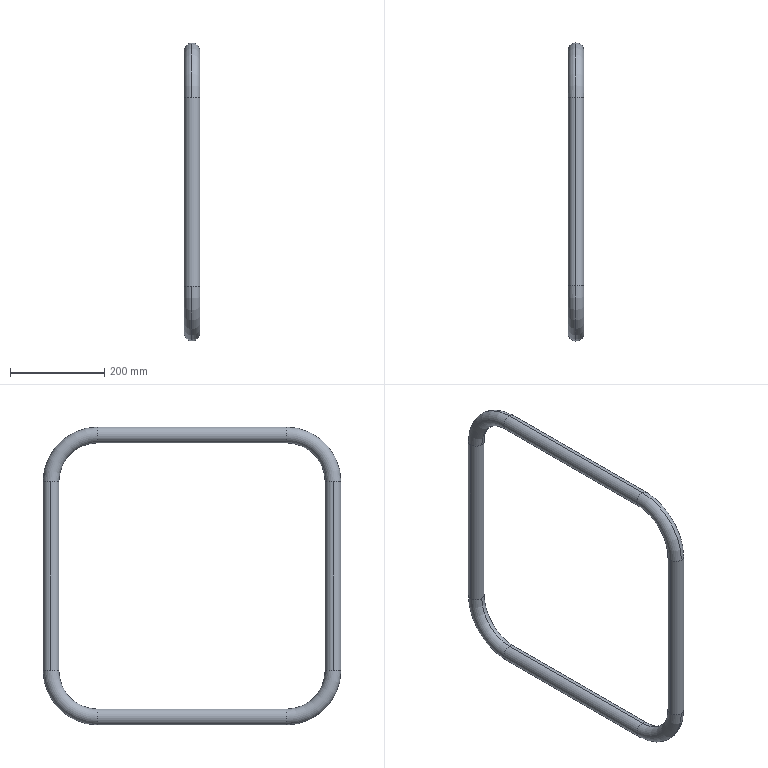Component | SolidWorks | Door-2 | 1 solid | 32 faces | box 33.5 x 633.5 x 633.5 mm | volume 640543 mm3 | torus 16 | cylinder 16 | commonest cylinder face diameters 33.5 x8 27.5 x8 | material Plain Carbon Steel
build123d program:
from build123d import *

# Parameters (mm, degrees)
SWEEP_THIN1_PROFILE_R   = 16.75
SWEEP_THIN1_PROFILE_R_2 = 13.75


with BuildPart() as part:
    # Sweep-Thin1: sweep along a path in Sketch1
    with BuildLine(Plane(origin=(0, 0, 0), x_dir=(0, 0, -1), z_dir=(1, 0, 0))) as sweep_thin1_path:
        Line((-438.875, 448.577), (-38.875, 448.577))
        ThreePointArc((-38.875, 448.577), (31.836, 419.288), (61.125, 348.577))
        Line((61.125, 348.577), (61.125, -51.423))
        ThreePointArc((61.125, -51.423), (31.836, -122.134), (-38.875, -151.423))
        Line((-38.875, -151.423), (-438.875, -151.423))
        ThreePointArc((-438.875, -151.423), (-509.586, -122.134), (-538.875, -51.423))
        Line((-538.875, -51.423), (-538.875, 348.577))
        ThreePointArc((-538.875, 348.577), (-509.586, 419.288), (-438.875, 448.577))
    # Sweep-Thin1 profile (on start of the path) → Sweep-Thin1 (sweep)
    with BuildSketch(Plane(origin=(0, 448.577, 438.875), x_dir=(-1, 0, 0), z_dir=(0, 0, -1))):
        Circle(SWEEP_THIN1_PROFILE_R)
        Circle(SWEEP_THIN1_PROFILE_R_2, mode=Mode.SUBTRACT)
    sweep(path=sweep_thin1_path.line)


solid = part.part

# Placed as in the assembly
solid = solid.moved(Location((-3322.199, 2439.746, 6247.098), (0, 0, 0)))
STEP:
#1=COLOUR_RGB('',0.7922,0.8196,0.9333);
#2=FILL_AREA_STYLE_COLOUR('',#1);
#3=FILL_AREA_STYLE('',(#2));
#4=SURFACE_STYLE_FILL_AREA(#3);
#5=SURFACE_SIDE_STYLE('',(#4));
#6=SURFACE_STYLE_USAGE(.BOTH.,#5);
#7=PRESENTATION_STYLE_ASSIGNMENT((#6));
#8=CARTESIAN_POINT('',(-130.795,89.432,263.227));
#9=VERTEX_POINT('',#8);
#10=CARTESIAN_POINT('',(-131.455,90.091,263.227));
#11=VERTEX_POINT('',#10);
#12=CARTESIAN_POINT('',(-130.795,90.091,263.227));
#13=DIRECTION('',(0.,0.,-1.));
#14=DIRECTION('',(0.,1.,0.));
#15=AXIS2_PLACEMENT_3D('',#12,#13,#14);
#16=CIRCLE('',#15,0.6594);
#17=EDGE_CURVE('',#9,#11,#16,.T.);
#18=ORIENTED_EDGE('',*,*,#17,.F.);
#19=CARTESIAN_POINT('',(-130.795,94.028,267.824));
#20=VERTEX_POINT('',#19);
#21=CARTESIAN_POINT('',(-130.795,94.028,263.227));
#22=DIRECTION('',(-1.,0.,0.));
#23=DIRECTION('',(0.,0.,1.));
#24=AXIS2_PLACEMENT_3D('',#21,#22,#23);
#25=CIRCLE('',#24,4.596);
#26=EDGE_CURVE('',#9,#20,#25,.T.);
#27=ORIENTED_EDGE('',*,*,#26,.T.);
#28=CARTESIAN_POINT('',(-130.795,94.028,266.505));
#29=VERTEX_POINT('',#28);
#30=CARTESIAN_POINT('',(-130.795,94.028,267.164));
#31=DIRECTION('',(0.,-1.,-0.));
#32=DIRECTION('',(0.,0.,-1.));
#33=AXIS2_PLACEMENT_3D('',#30,#31,#32);
#34=CIRCLE('',#33,0.6594);
#35=EDGE_CURVE('',#20,#29,#34,.T.);
#36=ORIENTED_EDGE('',*,*,#35,.T.);
#37=CARTESIAN_POINT('',(-130.795,90.751,263.227));
#38=VERTEX_POINT('',#37);
#39=CARTESIAN_POINT('',(-130.795,94.028,263.227));
#40=DIRECTION('',(-1.,0.,0.));
#41=DIRECTION('',(0.,0.,1.));
#42=AXIS2_PLACEMENT_3D('',#39,#40,#41);
#43=CIRCLE('',#42,3.278);
#44=EDGE_CURVE('',#38,#29,#43,.T.);
#45=ORIENTED_EDGE('',*,*,#44,.F.);
#46=CARTESIAN_POINT('',(-130.795,90.091,263.227));
#47=DIRECTION('',(0.,0.,-1.));
#48=DIRECTION('',(0.,1.,0.));
#49=AXIS2_PLACEMENT_3D('',#46,#47,#48);
#50=CIRCLE('',#49,0.6594);
#51=EDGE_CURVE('',#11,#38,#50,.T.);
#52=ORIENTED_EDGE('',*,*,#51,.F.);
#53=EDGE_LOOP('',(#18,#27,#36,#45,#52));
#54=FACE_OUTER_BOUND('',#53,.T.);
#55=CARTESIAN_POINT('',(-130.795,94.028,263.227));
#56=DIRECTION('',(-1.,0.,0.));
#57=DIRECTION('',(0.,0.,1.));
#58=AXIS2_PLACEMENT_3D('',#55,#56,#57);
#59=TOROIDAL_SURFACE('',#58,3.937,0.6594);
#60=ADVANCED_FACE('',(#54),#59,.T.);
#61=CARTESIAN_POINT('',(-130.795,94.028,242.883));
#62=VERTEX_POINT('',#61);
#63=CARTESIAN_POINT('',(-130.795,94.028,244.202));
#64=VERTEX_POINT('',#63);
#65=CARTESIAN_POINT('',(-130.795,94.028,243.542));
#66=DIRECTION('',(0.,1.,0.));
#67=DIRECTION('',(0.,0.,1.));
#68=AXIS2_PLACEMENT_3D('',#65,#66,#67);
#69=CIRCLE('',#68,0.6594);
#70=EDGE_CURVE('',#62,#64,#69,.T.);
#71=ORIENTED_EDGE('',*,*,#70,.F.);
#72=CARTESIAN_POINT('',(-130.795,89.432,247.479));
#73=VERTEX_POINT('',#72);
#74=CARTESIAN_POINT('',(-130.795,94.028,247.479));
#75=DIRECTION('',(-1.,0.,0.));
#76=DIRECTION('',(0.,0.,1.));
#77=AXIS2_PLACEMENT_3D('',#74,#75,#76);
#78=CIRCLE('',#77,4.596);
#79=EDGE_CURVE('',#62,#73,#78,.T.);
#80=ORIENTED_EDGE('',*,*,#79,.T.);
#81=CARTESIAN_POINT('',(-131.455,90.091,247.479));
#82=VERTEX_POINT('',#81);
#83=CARTESIAN_POINT('',(-130.795,90.091,247.479));
#84=DIRECTION('',(0.,0.,-1.));
#85=DIRECTION('',(0.,1.,0.));
#86=AXIS2_PLACEMENT_3D('',#83,#84,#85);
#87=CIRCLE('',#86,0.6594);
#88=EDGE_CURVE('',#73,#82,#87,.T.);
#89=ORIENTED_EDGE('',*,*,#88,.T.);
#90=CARTESIAN_POINT('',(-130.795,90.751,247.479));
#91=VERTEX_POINT('',#90);
#92=CARTESIAN_POINT('',(-130.795,90.091,247.479));
#93=DIRECTION('',(0.,0.,-1.));
#94=DIRECTION('',(0.,1.,0.));
#95=AXIS2_PLACEMENT_3D('',#92,#93,#94);
#96=CIRCLE('',#95,0.6594);
#97=EDGE_CURVE('',#82,#91,#96,.T.);
#98=ORIENTED_EDGE('',*,*,#97,.T.);
#99=CARTESIAN_POINT('',(-130.795,94.028,247.479));
#100=DIRECTION('',(-1.,0.,0.));
#101=DIRECTION('',(0.,0.,1.));
#102=AXIS2_PLACEMENT_3D('',#99,#100,#101);
#103=CIRCLE('',#102,3.278);
#104=EDGE_CURVE('',#64,#91,#103,.T.);
#105=ORIENTED_EDGE('',*,*,#104,.F.);
#106=EDGE_LOOP('',(#71,#80,#89,#98,#105));
#107=FACE_OUTER_BOUND('',#106,.T.);
#108=CARTESIAN_POINT('',(-130.795,94.028,247.479));
#109=DIRECTION('',(-1.,0.,0.));
#110=DIRECTION('',(0.,0.,1.));
#111=AXIS2_PLACEMENT_3D('',#108,#109,#110);
#112=TOROIDAL_SURFACE('',#111,3.937,0.6594);
#113=ADVANCED_FACE('',(#107),#112,.T.);
#114=CARTESIAN_POINT('',(-130.795,114.373,247.479));
#115=VERTEX_POINT('',#114);
#116=CARTESIAN_POINT('',(-131.455,113.713,247.479));
#117=VERTEX_POINT('',#116);
#118=CARTESIAN_POINT('',(-130.795,113.713,247.479));
#119=DIRECTION('',(0.,-0.,1.));
#120=DIRECTION('',(0.,-1.,0.));
#121=AXIS2_PLACEMENT_3D('',#118,#119,#120);
#122=CIRCLE('',#121,0.6594);
#123=EDGE_CURVE('',#115,#117,#122,.T.);
#124=ORIENTED_EDGE('',*,*,#123,.F.);
#125=CARTESIAN_POINT('',(-130.795,109.776,242.883));
#126=VERTEX_POINT('',#125);
#127=CARTESIAN_POINT('',(-130.795,109.776,247.479));
#128=DIRECTION('',(-1.,0.,0.));
#129=DIRECTION('',(0.,0.,1.));
#130=AXIS2_PLACEMENT_3D('',#127,#128,#129);
#131=CIRCLE('',#130,4.596);
#132=EDGE_CURVE('',#115,#126,#131,.T.);
#133=ORIENTED_EDGE('',*,*,#132,.T.);
#134=CARTESIAN_POINT('',(-130.795,109.776,244.202));
#135=VERTEX_POINT('',#134);
#136=CARTESIAN_POINT('',(-130.795,109.776,243.542));
#137=DIRECTION('',(0.,1.,0.));
#138=DIRECTION('',(0.,0.,1.));
#139=AXIS2_PLACEMENT_3D('',#136,#137,#138);
#140=CIRCLE('',#139,0.6594);
#141=EDGE_CURVE('',#126,#135,#140,.T.);
#142=ORIENTED_EDGE('',*,*,#141,.T.);
#143=CARTESIAN_POINT('',(-130.795,113.054,247.479));
#144=VERTEX_POINT('',#143);
#145=CARTESIAN_POINT('',(-130.795,109.776,247.479));
#146=DIRECTION('',(-1.,0.,0.));
#147=DIRECTION('',(0.,0.,1.));
#148=AXIS2_PLACEMENT_3D('',#145,#146,#147);
#149=CIRCLE('',#148,3.278);
#150=EDGE_CURVE('',#144,#135,#149,.T.);
#151=ORIENTED_EDGE('',*,*,#150,.F.);
#152=CARTESIAN_POINT('',(-130.795,113.713,247.479));
#153=DIRECTION('',(0.,-0.,1.));
#154=DIRECTION('',(0.,-1.,0.));
#155=AXIS2_PLACEMENT_3D('',#152,#153,#154);
#156=CIRCLE('',#155,0.6594);
#157=EDGE_CURVE('',#117,#144,#156,.T.);
#158=ORIENTED_EDGE('',*,*,#157,.F.);
#159=EDGE_LOOP('',(#124,#133,#142,#151,#158));
#160=FACE_OUTER_BOUND('',#159,.T.);
#161=CARTESIAN_POINT('',(-130.795,109.776,247.479));
#162=DIRECTION('',(-1.,0.,0.));
#163=DIRECTION('',(0.,0.,1.));
#164=AXIS2_PLACEMENT_3D('',#161,#162,#163);
#165=TOROIDAL_SURFACE('',#164,3.937,0.6594);
#166=ADVANCED_FACE('',(#160),#165,.T.);
#167=CARTESIAN_POINT('',(-130.795,109.776,267.824));
#168=VERTEX_POINT('',#167);
#169=CARTESIAN_POINT('',(-130.795,109.776,266.505));
#170=VERTEX_POINT('',#169);
#171=CARTESIAN_POINT('',(-130.795,109.776,267.164));
#172=DIRECTION('',(0.,-1.,-0.));
#173=DIRECTION('',(0.,0.,-1.));
#174=AXIS2_PLACEMENT_3D('',#171,#172,#173);
#175=CIRCLE('',#174,0.6594);
#176=EDGE_CURVE('',#168,#170,#175,.T.);
#177=ORIENTED_EDGE('',*,*,#176,.F.);
#178=CARTESIAN_POINT('',(-130.795,114.373,263.227));
#179=VERTEX_POINT('',#178);
#180=CARTESIAN_POINT('',(-130.795,109.776,263.227));
#181=DIRECTION('',(-1.,0.,0.));
#182=DIRECTION('',(0.,0.,1.));
#183=AXIS2_PLACEMENT_3D('',#180,#181,#182);
#184=CIRCLE('',#183,4.596);
#185=EDGE_CURVE('',#168,#179,#184,.T.);
#186=ORIENTED_EDGE('',*,*,#185,.T.);
#187=CARTESIAN_POINT('',(-131.455,113.713,263.227));
#188=VERTEX_POINT('',#187);
#189=CARTESIAN_POINT('',(-130.795,113.713,263.227));
#190=DIRECTION('',(0.,-0.,1.));
#191=DIRECTION('',(0.,-1.,0.));
#192=AXIS2_PLACEMENT_3D('',#189,#190,#191);
#193=CIRCLE('',#192,0.6594);
#194=EDGE_CURVE('',#179,#188,#193,.T.);
#195=ORIENTED_EDGE('',*,*,#194,.T.);
#196=CARTESIAN_POINT('',(-130.795,113.054,263.227));
#197=VERTEX_POINT('',#196);
#198=CARTESIAN_POINT('',(-130.795,113.713,263.227));
#199=DIRECTION('',(0.,-0.,1.));
#200=DIRECTION('',(0.,-1.,0.));
#201=AXIS2_PLACEMENT_3D('',#198,#199,#200);
#202=CIRCLE('',#201,0.6594);
#203=EDGE_CURVE('',#188,#197,#202,.T.);
#204=ORIENTED_EDGE('',*,*,#203,.T.);
#205=CARTESIAN_POINT('',(-130.795,109.776,263.227));
#206=DIRECTION('',(-1.,0.,0.));
#207=DIRECTION('',(0.,0.,1.));
#208=AXIS2_PLACEMENT_3D('',#205,#206,#207);
#209=CIRCLE('',#208,3.278);
#210=EDGE_CURVE('',#170,#197,#209,.T.);
#211=ORIENTED_EDGE('',*,*,#210,.F.);
#212=EDGE_LOOP('',(#177,#186,#195,#204,#211));
#213=FACE_OUTER_BOUND('',#212,.T.);
#214=CARTESIAN_POINT('',(-130.795,109.776,263.227));
#215=DIRECTION('',(-1.,0.,0.));
#216=DIRECTION('',(0.,0.,1.));
#217=AXIS2_PLACEMENT_3D('',#214,#215,#216);
#218=TOROIDAL_SURFACE('',#217,3.937,0.6594);
#219=ADVANCED_FACE('',(#213),#218,.T.);
#220=CARTESIAN_POINT('',(-130.795,94.028,267.164));
#221=DIRECTION('',(0.,-1.,-0.));
#222=DIRECTION('',(0.,0.,-1.));
#223=AXIS2_PLACEMENT_3D('',#220,#221,#222);
#224=CIRCLE('',#223,0.6594);
#225=EDGE_CURVE('',#29,#20,#224,.T.);
#226=ORIENTED_EDGE('',*,*,#225,.F.);
#227=CARTESIAN_POINT('',(-130.795,94.028,266.505));
#228=DIRECTION('',(0.,1.,0.));
#229=VECTOR('',#228,39.37);
#230=LINE('',#227,#229);
#231=EDGE_CURVE('',#29,#170,#230,.T.);
#232=ORIENTED_EDGE('',*,*,#231,.T.);
#233=CARTESIAN_POINT('',(-130.795,109.776,267.164));
#234=DIRECTION('',(0.,-1.,-0.));
#235=DIRECTION('',(0.,0.,-1.));
#236=AXIS2_PLACEMENT_3D('',#233,#234,#235);
#237=CIRCLE('',#236,0.6594);
#238=EDGE_CURVE('',#170,#168,#237,.T.);
#239=ORIENTED_EDGE('',*,*,#238,.T.);
#240=CARTESIAN_POINT('',(-130.795,94.028,267.824));
#241=DIRECTION('',(0.,1.,0.));
#242=VECTOR('',#241,39.37);
#243=LINE('',#240,#242);
#244=EDGE_CURVE('',#20,#168,#243,.T.);
#245=ORIENTED_EDGE('',*,*,#244,.F.);
#246=EDGE_LOOP('',(#226,#232,#239,#245));
#247=FACE_OUTER_BOUND('',#246,.T.);
#248=CARTESIAN_POINT('',(-130.795,94.028,267.164));
#249=DIRECTION('',(0.,1.,0.));
#250=DIRECTION('',(0.,0.,1.));
#251=AXIS2_PLACEMENT_3D('',#248,#249,#250);
#252=CYLINDRICAL_SURFACE('',#251,0.6594);
#253=ADVANCED_FACE('',(#247),#252,.T.);
#254=ORIENTED_EDGE('',*,*,#97,.F.);
#255=CARTESIAN_POINT('',(-131.455,90.091,247.479));
#256=DIRECTION('',(0.,0.,1.));
#257=VECTOR('',#256,39.37);
#258=LINE('',#255,#257);
#259=EDGE_CURVE('',#82,#11,#258,.T.);
#260=ORIENTED_EDGE('',*,*,#259,.T.);
#261=ORIENTED_EDGE('',*,*,#51,.T.);
#262=CARTESIAN_POINT('',(-130.136,90.091,263.227));
#263=VERTEX_POINT('',#262);
#264=CARTESIAN_POINT('',(-130.795,90.091,263.227));
#265=DIRECTION('',(0.,0.,-1.));
#266=DIRECTION('',(0.,1.,0.));
#267=AXIS2_PLACEMENT_3D('',#264,#265,#266);
#268=CIRCLE('',#267,0.6594);
#269=EDGE_CURVE('',#38,#263,#268,.T.);
#270=ORIENTED_EDGE('',*,*,#269,.T.);
#271=CARTESIAN_POINT('',(-130.136,90.091,247.479));
#272=VERTEX_POINT('',#271);
#273=CARTESIAN_POINT('',(-130.136,90.091,247.479));
#274=DIRECTION('',(0.,0.,1.));
#275=VECTOR('',#274,39.37);
#276=LINE('',#273,#275);
#277=EDGE_CURVE('',#272,#263,#276,.T.);
#278=ORIENTED_EDGE('',*,*,#277,.F.);
#279=CARTESIAN_POINT('',(-130.795,90.091,247.479));
#280=DIRECTION('',(0.,0.,-1.));
#281=DIRECTION('',(0.,1.,0.));
#282=AXIS2_PLACEMENT_3D('',#279,#280,#281);
#283=CIRCLE('',#282,0.6594);
#284=EDGE_CURVE('',#91,#272,#283,.T.);
#285=ORIENTED_EDGE('',*,*,#284,.F.);
#286=EDGE_LOOP('',(#254,#260,#261,#270,#278,#285));
#287=FACE_OUTER_BOUND('',#286,.T.);
#288=CARTESIAN_POINT('',(-130.795,90.091,247.479));
#289=DIRECTION('',(0.,0.,1.));
#290=DIRECTION('',(1.,0.,0.));
#291=AXIS2_PLACEMENT_3D('',#288,#289,#290);
#292=CYLINDRICAL_SURFACE('',#291,0.6594);
#293=ADVANCED_FACE('',(#287),#292,.T.);
#294=CARTESIAN_POINT('',(-130.795,109.776,243.542));
#295=DIRECTION('',(0.,1.,0.));
#296=DIRECTION('',(0.,0.,1.));
#297=AXIS2_PLACEMENT_3D('',#294,#295,#296);
#298=CIRCLE('',#297,0.6594);
#299=EDGE_CURVE('',#135,#126,#298,.T.);
#300=ORIENTED_EDGE('',*,*,#299,.F.);
#301=CARTESIAN_POINT('',(-130.795,109.776,244.202));
#302=DIRECTION('',(0.,-1.,-0.));
#303=VECTOR('',#302,39.37);
#304=LINE('',#301,#303);
#305=EDGE_CURVE('',#135,#64,#304,.T.);
#306=ORIENTED_EDGE('',*,*,#305,.T.);
#307=CARTESIAN_POINT('',(-130.795,94.028,243.542));
#308=DIRECTION('',(0.,1.,0.));
#309=DIRECTION('',(0.,0.,1.));
#310=AXIS2_PLACEMENT_3D('',#307,#308,#309);
#311=CIRCLE('',#310,0.6594);
#312=EDGE_CURVE('',#64,#62,#311,.T.);
#313=ORIENTED_EDGE('',*,*,#312,.T.);
#314=CARTESIAN_POINT('',(-130.795,109.776,242.883));
#315=DIRECTION('',(0.,-1.,-0.));
#316=VECTOR('',#315,39.37);
#317=LINE('',#314,#316);
#318=EDGE_CURVE('',#126,#62,#317,.T.);
#319=ORIENTED_EDGE('',*,*,#318,.F.);
#320=EDGE_LOOP('',(#300,#306,#313,#319));
#321=FACE_OUTER_BOUND('',#320,.T.);
#322=CARTESIAN_POINT('',(-130.795,109.776,243.542));
#323=DIRECTION('',(0.,-1.,-0.));
#324=DIRECTION('',(0.,0.,-1.));
#325=AXIS2_PLACEMENT_3D('',#322,#323,#324);
#326=CYLINDRICAL_SURFACE('',#325,0.6594);
#327=ADVANCED_FACE('',(#321),#326,.T.);
#328=CARTESIAN_POINT('',(-130.136,113.713,263.227));
#329=VERTEX_POINT('',#328);
#330=CARTESIAN_POINT('',(-130.795,113.713,263.227));
#331=DIRECTION('',(0.,-0.,1.));
#332=DIRECTION('',(0.,-1.,0.));
#333=AXIS2_PLACEMENT_3D('',#330,#331,#332);
#334=CIRCLE('',#333,0.6594);
#335=EDGE_CURVE('',#329,#179,#334,.T.);
#336=ORIENTED_EDGE('',*,*,#335,.F.);
#337=CARTESIAN_POINT('',(-130.136,113.713,247.479));
#338=VERTEX_POINT('',#337);
#339=CARTESIAN_POINT('',(-130.136,113.713,263.227));
#340=DIRECTION('',(0.,0.,-1.));
#341=VECTOR('',#340,39.37);
#342=LINE('',#339,#341);
#343=EDGE_CURVE('',#329,#338,#342,.T.);
#344=ORIENTED_EDGE('',*,*,#343,.T.);
#345=CARTESIAN_POINT('',(-130.795,113.713,247.479));
#346=DIRECTION('',(0.,-0.,1.));
#347=DIRECTION('',(0.,-1.,0.));
#348=AXIS2_PLACEMENT_3D('',#345,#346,#347);
#349=CIRCLE('',#348,0.6594);
#350=EDGE_CURVE('',#338,#115,#349,.T.);
#351=ORIENTED_EDGE('',*,*,#350,.T.);
#352=ORIENTED_EDGE('',*,*,#123,.T.);
#353=CARTESIAN_POINT('',(-131.455,113.713,263.227));
#354=DIRECTION('',(0.,0.,-1.));
#355=VECTOR('',#354,39.37);
#356=LINE('',#353,#355);
#357=EDGE_CURVE('',#188,#117,#356,.T.);
#358=ORIENTED_EDGE('',*,*,#357,.F.);
#359=ORIENTED_EDGE('',*,*,#194,.F.);
#360=EDGE_LOOP('',(#336,#344,#351,#352,#358,#359));
#361=FACE_OUTER_BOUND('',#360,.T.);
#362=CARTESIAN_POINT('',(-130.795,113.713,263.227));
#363=DIRECTION('',(0.,0.,-1.));
#364=DIRECTION('',(-1.,0.,0.));
#365=AXIS2_PLACEMENT_3D('',#362,#363,#364);
#366=CYLINDRICAL_SURFACE('',#365,0.6594);
#367=ADVANCED_FACE('',(#361),#366,.T.);
#368=ORIENTED_EDGE('',*,*,#185,.F.);
#369=ORIENTED_EDGE('',*,*,#238,.F.);
#370=ORIENTED_EDGE('',*,*,#210,.T.);
#371=CARTESIAN_POINT('',(-130.795,113.713,263.227));
#372=DIRECTION('',(0.,-0.,1.));
#373=DIRECTION('',(0.,-1.,0.));
#374=AXIS2_PLACEMENT_3D('',#371,#372,#373);
#375=CIRCLE('',#374,0.6594);
#376=EDGE_CURVE('',#197,#329,#375,.T.);
#377=ORIENTED_EDGE('',*,*,#376,.T.);
#378=ORIENTED_EDGE('',*,*,#335,.T.);
#379=EDGE_LOOP('',(#368,#369,#370,#377,#378));
#380=FACE_OUTER_BOUND('',#379,.T.);
#381=CARTESIAN_POINT('',(-130.795,109.776,263.227));
#382=DIRECTION('',(-1.,0.,0.));
#383=DIRECTION('',(0.,0.,1.));
#384=AXIS2_PLACEMENT_3D('',#381,#382,#383);
#385=TOROIDAL_SURFACE('',#384,3.937,0.6594);
#386=ADVANCED_FACE('',(#380),#385,.T.);
#387=ORIENTED_EDGE('',*,*,#343,.F.);
#388=ORIENTED_EDGE('',*,*,#376,.F.);
#389=ORIENTED_EDGE('',*,*,#203,.F.);
#390=ORIENTED_EDGE('',*,*,#357,.T.);
#391=ORIENTED_EDGE('',*,*,#157,.T.);
#392=CARTESIAN_POINT('',(-130.795,113.713,247.479));
#393=DIRECTION('',(0.,-0.,1.));
#394=DIRECTION('',(0.,-1.,0.));
#395=AXIS2_PLACEMENT_3D('',#392,#393,#394);
#396=CIRCLE('',#395,0.6594);
#397=EDGE_CURVE('',#144,#338,#396,.T.);
#398=ORIENTED_EDGE('',*,*,#397,.T.);
#399=EDGE_LOOP('',(#387,#388,#389,#390,#391,#398));
#400=FACE_OUTER_BOUND('',#399,.T.);
#401=CARTESIAN_POINT('',(-130.795,113.713,263.227));
#402=DIRECTION('',(0.,0.,-1.));
#403=DIRECTION('',(-1.,0.,0.));
#404=AXIS2_PLACEMENT_3D('',#401,#402,#403);
#405=CYLINDRICAL_SURFACE('',#404,0.6594);
#406=ADVANCED_FACE('',(#400),#405,.T.);
#407=ORIENTED_EDGE('',*,*,#132,.F.);
#408=ORIENTED_EDGE('',*,*,#350,.F.);
#409=ORIENTED_EDGE('',*,*,#397,.F.);
#410=ORIENTED_EDGE('',*,*,#150,.T.);
#411=ORIENTED_EDGE('',*,*,#299,.T.);
#412=EDGE_LOOP('',(#407,#408,#409,#410,#411));
#413=FACE_OUTER_BOUND('',#412,.T.);
#414=CARTESIAN_POINT('',(-130.795,109.776,247.479));
#415=DIRECTION('',(-1.,0.,0.));
#416=DIRECTION('',(0.,0.,1.));
#417=AXIS2_PLACEMENT_3D('',#414,#415,#416);
#418=TOROIDAL_SURFACE('',#417,3.937,0.6594);
#419=ADVANCED_FACE('',(#413),#418,.T.);
#420=ORIENTED_EDGE('',*,*,#305,.F.);
#421=ORIENTED_EDGE('',*,*,#141,.F.);
#422=ORIENTED_EDGE('',*,*,#318,.T.);
#423=ORIENTED_EDGE('',*,*,#70,.T.);
#424=EDGE_LOOP('',(#420,#421,#422,#423));
#425=FACE_OUTER_BOUND('',#424,.T.);
#426=CARTESIAN_POINT('',(-130.795,109.776,243.542));
#427=DIRECTION('',(0.,-1.,-0.));
#428=DIRECTION('',(0.,0.,-1.));
#429=AXIS2_PLACEMENT_3D('',#426,#427,#428);
#430=CYLINDRICAL_SURFACE('',#429,0.6594);
#431=ADVANCED_FACE('',(#425),#430,.T.);
#432=ORIENTED_EDGE('',*,*,#79,.F.);
#433=ORIENTED_EDGE('',*,*,#312,.F.);
#434=ORIENTED_EDGE('',*,*,#104,.T.);
#435=ORIENTED_EDGE('',*,*,#284,.T.);
#436=CARTESIAN_POINT('',(-130.795,90.091,247.479));
#437=DIRECTION('',(0.,0.,-1.));
#438=DIRECTION('',(0.,1.,0.));
#439=AXIS2_PLACEMENT_3D('',#436,#437,#438);
#440=CIRCLE('',#439,0.6594);
#441=EDGE_CURVE('',#272,#73,#440,.T.);
#442=ORIENTED_EDGE('',*,*,#441,.T.);
#443=EDGE_LOOP('',(#432,#433,#434,#435,#442));
#444=FACE_OUTER_BOUND('',#443,.T.);
#445=CARTESIAN_POINT('',(-130.795,94.028,247.479));
#446=DIRECTION('',(-1.,0.,0.));
#447=DIRECTION('',(0.,0.,1.));
#448=AXIS2_PLACEMENT_3D('',#445,#446,#447);
#449=TOROIDAL_SURFACE('',#448,3.937,0.6594);
#450=ADVANCED_FACE('',(#444),#449,.T.);
#451=ORIENTED_EDGE('',*,*,#259,.F.);
#452=ORIENTED_EDGE('',*,*,#88,.F.);
#453=ORIENTED_EDGE('',*,*,#441,.F.);
#454=ORIENTED_EDGE('',*,*,#277,.T.);
#455=CARTESIAN_POINT('',(-130.795,90.091,263.227));
#456=DIRECTION('',(0.,0.,-1.));
#457=DIRECTION('',(0.,1.,0.));
#458=AXIS2_PLACEMENT_3D('',#455,#456,#457);
#459=CIRCLE('',#458,0.6594);
#460=EDGE_CURVE('',#263,#9,#459,.T.);
#461=ORIENTED_EDGE('',*,*,#460,.T.);
#462=ORIENTED_EDGE('',*,*,#17,.T.);
#463=EDGE_LOOP('',(#451,#452,#453,#454,#461,#462));
#464=FACE_OUTER_BOUND('',#463,.T.);
#465=CARTESIAN_POINT('',(-130.795,90.091,247.479));
#466=DIRECTION('',(0.,0.,1.));
#467=DIRECTION('',(1.,0.,0.));
#468=AXIS2_PLACEMENT_3D('',#465,#466,#467);
#469=CYLINDRICAL_SURFACE('',#468,0.6594);
#470=ADVANCED_FACE('',(#464),#469,.T.);
#471=ORIENTED_EDGE('',*,*,#26,.F.);
#472=ORIENTED_EDGE('',*,*,#460,.F.);
#473=ORIENTED_EDGE('',*,*,#269,.F.);
#474=ORIENTED_EDGE('',*,*,#44,.T.);
#475=ORIENTED_EDGE('',*,*,#225,.T.);
#476=EDGE_LOOP('',(#471,#472,#473,#474,#475));
#477=FACE_OUTER_BOUND('',#476,.T.);
#478=CARTESIAN_POINT('',(-130.795,94.028,263.227));
#479=DIRECTION('',(-1.,0.,0.));
#480=DIRECTION('',(0.,0.,1.));
#481=AXIS2_PLACEMENT_3D('',#478,#479,#480);
#482=TOROIDAL_SURFACE('',#481,3.937,0.6594);
#483=ADVANCED_FACE('',(#477),#482,.T.);
#484=ORIENTED_EDGE('',*,*,#231,.F.);
#485=ORIENTED_EDGE('',*,*,#35,.F.);
#486=ORIENTED_EDGE('',*,*,#244,.T.);
#487=ORIENTED_EDGE('',*,*,#176,.T.);
#488=EDGE_LOOP('',(#484,#485,#486,#487));
#489=FACE_OUTER_BOUND('',#488,.T.);
#490=CARTESIAN_POINT('',(-130.795,94.028,267.164));
#491=DIRECTION('',(0.,1.,0.));
#492=DIRECTION('',(0.,0.,1.));
#493=AXIS2_PLACEMENT_3D('',#490,#491,#492);
#494=CYLINDRICAL_SURFACE('',#493,0.6594);
#495=ADVANCED_FACE('',(#489),#494,.T.);
#496=CLOSED_SHELL('',(#60,#113,#166,#219,#253,#293,#327,#367,#386,#406,#419,#431,#450,#470,#483,#495));
#497=CARTESIAN_POINT('',(-130.254,90.091,263.227));
#498=VERTEX_POINT('',#497);
#499=CARTESIAN_POINT('',(-130.795,89.55,263.227));
#500=VERTEX_POINT('',#499);
#501=CARTESIAN_POINT('',(-130.795,90.091,263.227));
#502=DIRECTION('',(0.,0.,-1.));
#503=DIRECTION('',(1.,0.,0.));
#504=AXIS2_PLACEMENT_3D('',#501,#502,#503);
#505=CIRCLE('',#504,0.5413);
#506=EDGE_CURVE('',#498,#500,#505,.T.);
#507=ORIENTED_EDGE('',*,*,#506,.T.);
#508=CARTESIAN_POINT('',(-130.795,94.028,267.706));
#509=VERTEX_POINT('',#508);
#510=CARTESIAN_POINT('',(-130.795,94.028,263.227));
#511=DIRECTION('',(-1.,0.,0.));
#512=DIRECTION('',(0.,0.,1.));
#513=AXIS2_PLACEMENT_3D('',#510,#511,#512);
#514=CIRCLE('',#513,4.478);
#515=EDGE_CURVE('',#500,#509,#514,.T.);
#516=ORIENTED_EDGE('',*,*,#515,.T.);
#517=CARTESIAN_POINT('',(-130.795,94.028,266.623));
#518=VERTEX_POINT('',#517);
#519=CARTESIAN_POINT('',(-130.795,94.028,267.164));
#520=DIRECTION('',(0.,-1.,0.));
#521=DIRECTION('',(0.,0.,-1.));
#522=AXIS2_PLACEMENT_3D('',#519,#520,#521);
#523=CIRCLE('',#522,0.5413);
#524=EDGE_CURVE('',#518,#509,#523,.T.);
#525=ORIENTED_EDGE('',*,*,#524,.F.);
#526=CARTESIAN_POINT('',(-130.795,90.633,263.227));
#527=VERTEX_POINT('',#526);
#528=CARTESIAN_POINT('',(-130.795,94.028,263.227));
#529=DIRECTION('',(-1.,0.,0.));
#530=DIRECTION('',(0.,0.,1.));
#531=AXIS2_PLACEMENT_3D('',#528,#529,#530);
#532=CIRCLE('',#531,3.396);
#533=EDGE_CURVE('',#527,#518,#532,.T.);
#534=ORIENTED_EDGE('',*,*,#533,.F.);
#535=CARTESIAN_POINT('',(-130.795,90.091,263.227));
#536=DIRECTION('',(0.,0.,-1.));
#537=DIRECTION('',(1.,0.,0.));
#538=AXIS2_PLACEMENT_3D('',#535,#536,#537);
#539=CIRCLE('',#538,0.5413);
#540=EDGE_CURVE('',#527,#498,#539,.T.);
#541=ORIENTED_EDGE('',*,*,#540,.T.);
#542=EDGE_LOOP('',(#507,#516,#525,#534,#541));
#543=FACE_OUTER_BOUND('',#542,.T.);
#544=CARTESIAN_POINT('',(-130.795,94.028,263.227));
#545=DIRECTION('',(-1.,0.,0.));
#546=DIRECTION('',(0.,0.,1.));
#547=AXIS2_PLACEMENT_3D('',#544,#545,#546);
#548=TOROIDAL_SURFACE('',#547,3.937,0.5413);
#549=ADVANCED_FACE('',(#543),#548,.F.);
#550=CARTESIAN_POINT('',(-130.795,94.028,244.084));
#551=VERTEX_POINT('',#550);
#552=CARTESIAN_POINT('',(-130.795,94.028,243.001));
#553=VERTEX_POINT('',#552);
#554=CARTESIAN_POINT('',(-130.795,94.028,243.542));
#555=DIRECTION('',(0.,1.,0.));
#556=DIRECTION('',(0.,0.,-1.));
#557=AXIS2_PLACEMENT_3D('',#554,#555,#556);
#558=CIRCLE('',#557,0.5413);
#559=EDGE_CURVE('',#551,#553,#558,.T.);
#560=ORIENTED_EDGE('',*,*,#559,.T.);
#561=CARTESIAN_POINT('',(-130.795,89.55,247.479));
#562=VERTEX_POINT('',#561);
#563=CARTESIAN_POINT('',(-130.795,94.028,247.479));
#564=DIRECTION('',(-1.,0.,0.));
#565=DIRECTION('',(0.,0.,1.));
#566=AXIS2_PLACEMENT_3D('',#563,#564,#565);
#567=CIRCLE('',#566,4.478);
#568=EDGE_CURVE('',#553,#562,#567,.T.);
#569=ORIENTED_EDGE('',*,*,#568,.T.);
#570=CARTESIAN_POINT('',(-130.254,90.091,247.479));
#571=VERTEX_POINT('',#570);
#572=CARTESIAN_POINT('',(-130.795,90.091,247.479));
#573=DIRECTION('',(0.,0.,-1.));
#574=DIRECTION('',(0.,1.,0.));
#575=AXIS2_PLACEMENT_3D('',#572,#573,#574);
#576=CIRCLE('',#575,0.5413);
#577=EDGE_CURVE('',#571,#562,#576,.T.);
#578=ORIENTED_EDGE('',*,*,#577,.F.);
#579=CARTESIAN_POINT('',(-130.795,90.633,247.479));
#580=VERTEX_POINT('',#579);
#581=CARTESIAN_POINT('',(-130.795,90.091,247.479));
#582=DIRECTION('',(0.,0.,-1.));
#583=DIRECTION('',(0.,1.,0.));
#584=AXIS2_PLACEMENT_3D('',#581,#582,#583);
#585=CIRCLE('',#584,0.5413);
#586=EDGE_CURVE('',#580,#571,#585,.T.);
#587=ORIENTED_EDGE('',*,*,#586,.F.);
#588=CARTESIAN_POINT('',(-130.795,94.028,247.479));
#589=DIRECTION('',(-1.,0.,0.));
#590=DIRECTION('',(0.,0.,1.));
#591=AXIS2_PLACEMENT_3D('',#588,#589,#590);
#592=CIRCLE('',#591,3.396);
#593=EDGE_CURVE('',#551,#580,#592,.T.);
#594=ORIENTED_EDGE('',*,*,#593,.F.);
#595=EDGE_LOOP('',(#560,#569,#578,#587,#594));
#596=FACE_OUTER_BOUND('',#595,.T.);
#597=CARTESIAN_POINT('',(-130.795,94.028,247.479));
#598=DIRECTION('',(-1.,0.,0.));
#599=DIRECTION('',(0.,0.,1.));
#600=AXIS2_PLACEMENT_3D('',#597,#598,#599);
#601=TOROIDAL_SURFACE('',#600,3.937,0.5413);
#602=ADVANCED_FACE('',(#596),#601,.F.);
#603=CARTESIAN_POINT('',(-130.254,113.713,247.479));
#604=VERTEX_POINT('',#603);
#605=CARTESIAN_POINT('',(-130.795,114.255,247.479));
#606=VERTEX_POINT('',#605);
#607=CARTESIAN_POINT('',(-130.795,113.713,247.479));
#608=DIRECTION('',(0.,0.,1.));
#609=DIRECTION('',(-1.,0.,0.));
#610=AXIS2_PLACEMENT_3D('',#607,#608,#609);
#611=CIRCLE('',#610,0.5413);
#612=EDGE_CURVE('',#604,#606,#611,.T.);
#613=ORIENTED_EDGE('',*,*,#612,.T.);
#614=CARTESIAN_POINT('',(-130.795,109.776,243.001));
#615=VERTEX_POINT('',#614);
#616=CARTESIAN_POINT('',(-130.795,109.776,247.479));
#617=DIRECTION('',(-1.,0.,0.));
#618=DIRECTION('',(0.,0.,1.));
#619=AXIS2_PLACEMENT_3D('',#616,#617,#618);
#620=CIRCLE('',#619,4.478);
#621=EDGE_CURVE('',#606,#615,#620,.T.);
#622=ORIENTED_EDGE('',*,*,#621,.T.);
#623=CARTESIAN_POINT('',(-130.795,109.776,244.084));
#624=VERTEX_POINT('',#623);
#625=CARTESIAN_POINT('',(-130.795,109.776,243.542));
#626=DIRECTION('',(0.,1.,0.));
#627=DIRECTION('',(0.,0.,1.));
#628=AXIS2_PLACEMENT_3D('',#625,#626,#627);
#629=CIRCLE('',#628,0.5413);
#630=EDGE_CURVE('',#624,#615,#629,.T.);
#631=ORIENTED_EDGE('',*,*,#630,.F.);
#632=CARTESIAN_POINT('',(-130.795,113.172,247.479));
#633=VERTEX_POINT('',#632);
#634=CARTESIAN_POINT('',(-130.795,109.776,247.479));
#635=DIRECTION('',(-1.,0.,0.));
#636=DIRECTION('',(0.,0.,1.));
#637=AXIS2_PLACEMENT_3D('',#634,#635,#636);
#638=CIRCLE('',#637,3.396);
#639=EDGE_CURVE('',#633,#624,#638,.T.);
#640=ORIENTED_EDGE('',*,*,#639,.F.);
#641=CARTESIAN_POINT('',(-130.795,113.713,247.479));
#642=DIRECTION('',(0.,0.,1.));
#643=DIRECTION('',(-1.,0.,0.));
#644=AXIS2_PLACEMENT_3D('',#641,#642,#643);
#645=CIRCLE('',#644,0.5413);
#646=EDGE_CURVE('',#633,#604,#645,.T.);
#647=ORIENTED_EDGE('',*,*,#646,.T.);
#648=EDGE_LOOP('',(#613,#622,#631,#640,#647));
#649=FACE_OUTER_BOUND('',#648,.T.);
#650=CARTESIAN_POINT('',(-130.795,109.776,247.479));
#651=DIRECTION('',(-1.,0.,0.));
#652=DIRECTION('',(0.,0.,1.));
#653=AXIS2_PLACEMENT_3D('',#650,#651,#652);
#654=TOROIDAL_SURFACE('',#653,3.937,0.5413);
#655=ADVANCED_FACE('',(#649),#654,.F.);
#656=CARTESIAN_POINT('',(-130.795,109.776,266.623));
#657=VERTEX_POINT('',#656);
#658=CARTESIAN_POINT('',(-130.795,109.776,267.706));
#659=VERTEX_POINT('',#658);
#660=CARTESIAN_POINT('',(-130.795,109.776,267.164));
#661=DIRECTION('',(0.,-1.,0.));
#662=DIRECTION('',(0.,0.,1.));
#663=AXIS2_PLACEMENT_3D('',#660,#661,#662);
#664=CIRCLE('',#663,0.5413);
#665=EDGE_CURVE('',#657,#659,#664,.T.);
#666=ORIENTED_EDGE('',*,*,#665,.T.);
#667=CARTESIAN_POINT('',(-130.795,114.255,263.227));
#668=VERTEX_POINT('',#667);
#669=CARTESIAN_POINT('',(-130.795,109.776,263.227));
#670=DIRECTION('',(-1.,0.,0.));
#671=DIRECTION('',(0.,0.,1.));
#672=AXIS2_PLACEMENT_3D('',#669,#670,#671);
#673=CIRCLE('',#672,4.478);
#674=EDGE_CURVE('',#659,#668,#673,.T.);
#675=ORIENTED_EDGE('',*,*,#674,.T.);
#676=CARTESIAN_POINT('',(-130.254,113.713,263.227));
#677=VERTEX_POINT('',#676);
#678=CARTESIAN_POINT('',(-130.795,113.713,263.227));
#679=DIRECTION('',(0.,-0.,1.));
#680=DIRECTION('',(0.,-1.,0.));
#681=AXIS2_PLACEMENT_3D('',#678,#679,#680);
#682=CIRCLE('',#681,0.5413);
#683=EDGE_CURVE('',#677,#668,#682,.T.);
#684=ORIENTED_EDGE('',*,*,#683,.F.);
#685=CARTESIAN_POINT('',(-130.795,113.172,263.227));
#686=VERTEX_POINT('',#685);
#687=CARTESIAN_POINT('',(-130.795,113.713,263.227));
#688=DIRECTION('',(0.,-0.,1.));
#689=DIRECTION('',(0.,-1.,0.));
#690=AXIS2_PLACEMENT_3D('',#687,#688,#689);
#691=CIRCLE('',#690,0.5413);
#692=EDGE_CURVE('',#686,#677,#691,.T.);
#693=ORIENTED_EDGE('',*,*,#692,.F.);
#694=CARTESIAN_POINT('',(-130.795,109.776,263.227));
#695=DIRECTION('',(-1.,0.,0.));
#696=DIRECTION('',(0.,0.,1.));
#697=AXIS2_PLACEMENT_3D('',#694,#695,#696);
#698=CIRCLE('',#697,3.396);
#699=EDGE_CURVE('',#657,#686,#698,.T.);
#700=ORIENTED_EDGE('',*,*,#699,.F.);
#701=EDGE_LOOP('',(#666,#675,#684,#693,#700));
#702=FACE_OUTER_BOUND('',#701,.T.);
#703=CARTESIAN_POINT('',(-130.795,109.776,263.227));
#704=DIRECTION('',(-1.,0.,0.));
#705=DIRECTION('',(0.,0.,1.));
#706=AXIS2_PLACEMENT_3D('',#703,#704,#705);
#707=TOROIDAL_SURFACE('',#706,3.937,0.5413);
#708=ADVANCED_FACE('',(#702),#707,.F.);
#709=CARTESIAN_POINT('',(-130.795,94.028,267.164));
#710=DIRECTION('',(0.,-1.,0.));
#711=DIRECTION('',(0.,0.,-1.));
#712=AXIS2_PLACEMENT_3D('',#709,#710,#711);
#713=CIRCLE('',#712,0.5413);
#714=EDGE_CURVE('',#509,#518,#713,.T.);
#715=ORIENTED_EDGE('',*,*,#714,.T.);
#716=CARTESIAN_POINT('',(-130.795,94.028,266.623));
#717=DIRECTION('',(0.,1.,0.));
#718=VECTOR('',#717,39.37);
#719=LINE('',#716,#718);
#720=EDGE_CURVE('',#518,#657,#719,.T.);
#721=ORIENTED_EDGE('',*,*,#720,.T.);
#722=CARTESIAN_POINT('',(-130.795,109.776,267.164));
#723=DIRECTION('',(0.,-1.,0.));
#724=DIRECTION('',(0.,0.,1.));
#725=AXIS2_PLACEMENT_3D('',#722,#723,#724);
#726=CIRCLE('',#725,0.5413);
#727=EDGE_CURVE('',#659,#657,#726,.T.);
#728=ORIENTED_EDGE('',*,*,#727,.F.);
#729=CARTESIAN_POINT('',(-130.795,94.028,267.706));
#730=DIRECTION('',(0.,1.,0.));
#731=VECTOR('',#730,39.37);
#732=LINE('',#729,#731);
#733=EDGE_CURVE('',#509,#659,#732,.T.);
#734=ORIENTED_EDGE('',*,*,#733,.F.);
#735=EDGE_LOOP('',(#715,#721,#728,#734));
#736=FACE_OUTER_BOUND('',#735,.T.);
#737=CARTESIAN_POINT('',(-130.795,94.028,267.164));
#738=DIRECTION('',(0.,1.,0.));
#739=DIRECTION('',(0.,0.,1.));
#740=AXIS2_PLACEMENT_3D('',#737,#738,#739);
#741=CYLINDRICAL_SURFACE('',#740,0.5413);
#742=ADVANCED_FACE('',(#736),#741,.F.);
#743=ORIENTED_EDGE('',*,*,#577,.T.);
#744=CARTESIAN_POINT('',(-131.337,90.091,247.479));
#745=VERTEX_POINT('',#744);
#746=CARTESIAN_POINT('',(-130.795,90.091,247.479));
#747=DIRECTION('',(0.,0.,-1.));
#748=DIRECTION('',(0.,1.,0.));
#749=AXIS2_PLACEMENT_3D('',#746,#747,#748);
#750=CIRCLE('',#749,0.5413);
#751=EDGE_CURVE('',#562,#745,#750,.T.);
#752=ORIENTED_EDGE('',*,*,#751,.T.);
#753=CARTESIAN_POINT('',(-131.337,90.091,263.227));
#754=VERTEX_POINT('',#753);
#755=CARTESIAN_POINT('',(-131.337,90.091,247.479));
#756=DIRECTION('',(0.,0.,1.));
#757=VECTOR('',#756,39.37);
#758=LINE('',#755,#757);
#759=EDGE_CURVE('',#745,#754,#758,.T.);
#760=ORIENTED_EDGE('',*,*,#759,.T.);
#761=CARTESIAN_POINT('',(-130.795,90.091,263.227));
#762=DIRECTION('',(0.,0.,-1.));
#763=DIRECTION('',(1.,0.,0.));
#764=AXIS2_PLACEMENT_3D('',#761,#762,#763);
#765=CIRCLE('',#764,0.5413);
#766=EDGE_CURVE('',#500,#754,#765,.T.);
#767=ORIENTED_EDGE('',*,*,#766,.F.);
#768=ORIENTED_EDGE('',*,*,#506,.F.);
#769=CARTESIAN_POINT('',(-130.254,90.091,247.479));
#770=DIRECTION('',(0.,0.,1.));
#771=VECTOR('',#770,39.37);
#772=LINE('',#769,#771);
#773=EDGE_CURVE('',#571,#498,#772,.T.);
#774=ORIENTED_EDGE('',*,*,#773,.F.);
#775=EDGE_LOOP('',(#743,#752,#760,#767,#768,#774));
#776=FACE_OUTER_BOUND('',#775,.T.);
#777=CARTESIAN_POINT('',(-130.795,90.091,247.479));
#778=DIRECTION('',(0.,0.,1.));
#779=DIRECTION('',(1.,0.,0.));
#780=AXIS2_PLACEMENT_3D('',#777,#778,#779);
#781=CYLINDRICAL_SURFACE('',#780,0.5413);
#782=ADVANCED_FACE('',(#776),#781,.F.);
#783=CARTESIAN_POINT('',(-130.795,109.776,243.542));
#784=DIRECTION('',(0.,1.,0.));
#785=DIRECTION('',(0.,0.,1.));
#786=AXIS2_PLACEMENT_3D('',#783,#784,#785);
#787=CIRCLE('',#786,0.5413);
#788=EDGE_CURVE('',#615,#624,#787,.T.);
#789=ORIENTED_EDGE('',*,*,#788,.T.);
#790=CARTESIAN_POINT('',(-130.795,109.776,244.084));
#791=DIRECTION('',(0.,-1.,-0.));
#792=VECTOR('',#791,39.37);
#793=LINE('',#790,#792);
#794=EDGE_CURVE('',#624,#551,#793,.T.);
#795=ORIENTED_EDGE('',*,*,#794,.T.);
#796=CARTESIAN_POINT('',(-130.795,94.028,243.542));
#797=DIRECTION('',(0.,1.,0.));
#798=DIRECTION('',(0.,0.,-1.));
#799=AXIS2_PLACEMENT_3D('',#796,#797,#798);
#800=CIRCLE('',#799,0.5413);
#801=EDGE_CURVE('',#553,#551,#800,.T.);
#802=ORIENTED_EDGE('',*,*,#801,.F.);
#803=CARTESIAN_POINT('',(-130.795,109.776,243.001));
#804=DIRECTION('',(0.,-1.,-0.));
#805=VECTOR('',#804,39.37);
#806=LINE('',#803,#805);
#807=EDGE_CURVE('',#615,#553,#806,.T.);
#808=ORIENTED_EDGE('',*,*,#807,.F.);
#809=EDGE_LOOP('',(#789,#795,#802,#808));
#810=FACE_OUTER_BOUND('',#809,.T.);
#811=CARTESIAN_POINT('',(-130.795,109.776,243.542));
#812=DIRECTION('',(0.,-1.,-0.));
#813=DIRECTION('',(0.,0.,-1.));
#814=AXIS2_PLACEMENT_3D('',#811,#812,#813);
#815=CYLINDRICAL_SURFACE('',#814,0.5413);
#816=ADVANCED_FACE('',(#810),#815,.F.);
#817=CARTESIAN_POINT('',(-131.337,113.713,263.227));
#818=VERTEX_POINT('',#817);
#819=CARTESIAN_POINT('',(-130.795,113.713,263.227));
#820=DIRECTION('',(0.,-0.,1.));
#821=DIRECTION('',(0.,-1.,0.));
#822=AXIS2_PLACEMENT_3D('',#819,#820,#821);
#823=CIRCLE('',#822,0.5413);
#824=EDGE_CURVE('',#818,#686,#823,.T.);
#825=ORIENTED_EDGE('',*,*,#824,.T.);
#826=ORIENTED_EDGE('',*,*,#692,.T.);
#827=CARTESIAN_POINT('',(-130.254,113.713,263.227));
#828=DIRECTION('',(0.,0.,-1.));
#829=VECTOR('',#828,39.37);
#830=LINE('',#827,#829);
#831=EDGE_CURVE('',#677,#604,#830,.T.);
#832=ORIENTED_EDGE('',*,*,#831,.T.);
#833=ORIENTED_EDGE('',*,*,#646,.F.);
#834=CARTESIAN_POINT('',(-131.337,113.713,247.479));
#835=VERTEX_POINT('',#834);
#836=CARTESIAN_POINT('',(-130.795,113.713,247.479));
#837=DIRECTION('',(0.,0.,1.));
#838=DIRECTION('',(-1.,0.,0.));
#839=AXIS2_PLACEMENT_3D('',#836,#837,#838);
#840=CIRCLE('',#839,0.5413);
#841=EDGE_CURVE('',#835,#633,#840,.T.);
#842=ORIENTED_EDGE('',*,*,#841,.F.);
#843=CARTESIAN_POINT('',(-131.337,113.713,263.227));
#844=DIRECTION('',(0.,0.,-1.));
#845=VECTOR('',#844,39.37);
#846=LINE('',#843,#845);
#847=EDGE_CURVE('',#818,#835,#846,.T.);
#848=ORIENTED_EDGE('',*,*,#847,.F.);
#849=EDGE_LOOP('',(#825,#826,#832,#833,#842,#848));
#850=FACE_OUTER_BOUND('',#849,.T.);
#851=CARTESIAN_POINT('',(-130.795,113.713,263.227));
#852=DIRECTION('',(0.,0.,-1.));
#853=DIRECTION('',(-1.,0.,0.));
#854=AXIS2_PLACEMENT_3D('',#851,#852,#853);
#855=CYLINDRICAL_SURFACE('',#854,0.5413);
#856=ADVANCED_FACE('',(#850),#855,.F.);
#857=ORIENTED_EDGE('',*,*,#674,.F.);
#858=ORIENTED_EDGE('',*,*,#727,.T.);
#859=ORIENTED_EDGE('',*,*,#699,.T.);
#860=ORIENTED_EDGE('',*,*,#824,.F.);
#861=CARTESIAN_POINT('',(-130.795,113.713,263.227));
#862=DIRECTION('',(0.,-0.,1.));
#863=DIRECTION('',(0.,-1.,0.));
#864=AXIS2_PLACEMENT_3D('',#861,#862,#863);
#865=CIRCLE('',#864,0.5413);
#866=EDGE_CURVE('',#668,#818,#865,.T.);
#867=ORIENTED_EDGE('',*,*,#866,.F.);
#868=EDGE_LOOP('',(#857,#858,#859,#860,#867));
#869=FACE_OUTER_BOUND('',#868,.T.);
#870=CARTESIAN_POINT('',(-130.795,109.776,263.227));
#871=DIRECTION('',(-1.,0.,0.));
#872=DIRECTION('',(0.,0.,1.));
#873=AXIS2_PLACEMENT_3D('',#870,#871,#872);
#874=TOROIDAL_SURFACE('',#873,3.937,0.5413);
#875=ADVANCED_FACE('',(#869),#874,.F.);
#876=ORIENTED_EDGE('',*,*,#831,.F.);
#877=ORIENTED_EDGE('',*,*,#683,.T.);
#878=ORIENTED_EDGE('',*,*,#866,.T.);
#879=ORIENTED_EDGE('',*,*,#847,.T.);
#880=CARTESIAN_POINT('',(-130.795,113.713,247.479));
#881=DIRECTION('',(0.,0.,1.));
#882=DIRECTION('',(-1.,0.,0.));
#883=AXIS2_PLACEMENT_3D('',#880,#881,#882);
#884=CIRCLE('',#883,0.5413);
#885=EDGE_CURVE('',#606,#835,#884,.T.);
#886=ORIENTED_EDGE('',*,*,#885,.F.);
#887=ORIENTED_EDGE('',*,*,#612,.F.);
#888=EDGE_LOOP('',(#876,#877,#878,#879,#886,#887));
#889=FACE_OUTER_BOUND('',#888,.T.);
#890=CARTESIAN_POINT('',(-130.795,113.713,263.227));
#891=DIRECTION('',(0.,0.,-1.));
#892=DIRECTION('',(-1.,0.,0.));
#893=AXIS2_PLACEMENT_3D('',#890,#891,#892);
#894=CYLINDRICAL_SURFACE('',#893,0.5413);
#895=ADVANCED_FACE('',(#889),#894,.F.);
#896=ORIENTED_EDGE('',*,*,#621,.F.);
#897=ORIENTED_EDGE('',*,*,#885,.T.);
#898=ORIENTED_EDGE('',*,*,#841,.T.);
#899=ORIENTED_EDGE('',*,*,#639,.T.);
#900=ORIENTED_EDGE('',*,*,#788,.F.);
#901=EDGE_LOOP('',(#896,#897,#898,#899,#900));
#902=FACE_OUTER_BOUND('',#901,.T.);
#903=CARTESIAN_POINT('',(-130.795,109.776,247.479));
#904=DIRECTION('',(-1.,0.,0.));
#905=DIRECTION('',(0.,0.,1.));
#906=AXIS2_PLACEMENT_3D('',#903,#904,#905);
#907=TOROIDAL_SURFACE('',#906,3.937,0.5413);
#908=ADVANCED_FACE('',(#902),#907,.F.);
#909=ORIENTED_EDGE('',*,*,#794,.F.);
#910=ORIENTED_EDGE('',*,*,#630,.T.);
#911=ORIENTED_EDGE('',*,*,#807,.T.);
#912=ORIENTED_EDGE('',*,*,#559,.F.);
#913=EDGE_LOOP('',(#909,#910,#911,#912));
#914=FACE_OUTER_BOUND('',#913,.T.);
#915=CARTESIAN_POINT('',(-130.795,109.776,243.542));
#916=DIRECTION('',(0.,-1.,-0.));
#917=DIRECTION('',(0.,0.,-1.));
#918=AXIS2_PLACEMENT_3D('',#915,#916,#917);
#919=CYLINDRICAL_SURFACE('',#918,0.5413);
#920=ADVANCED_FACE('',(#914),#919,.F.);
#921=ORIENTED_EDGE('',*,*,#568,.F.);
#922=ORIENTED_EDGE('',*,*,#801,.T.);
#923=ORIENTED_EDGE('',*,*,#593,.T.);
#924=CARTESIAN_POINT('',(-130.795,90.091,247.479));
#925=DIRECTION('',(0.,0.,-1.));
#926=DIRECTION('',(0.,1.,0.));
#927=AXIS2_PLACEMENT_3D('',#924,#925,#926);
#928=CIRCLE('',#927,0.5413);
#929=EDGE_CURVE('',#745,#580,#928,.T.);
#930=ORIENTED_EDGE('',*,*,#929,.F.);
#931=ORIENTED_EDGE('',*,*,#751,.F.);
#932=EDGE_LOOP('',(#921,#922,#923,#930,#931));
#933=FACE_OUTER_BOUND('',#932,.T.);
#934=CARTESIAN_POINT('',(-130.795,94.028,247.479));
#935=DIRECTION('',(-1.,0.,0.));
#936=DIRECTION('',(0.,0.,1.));
#937=AXIS2_PLACEMENT_3D('',#934,#935,#936);
#938=TOROIDAL_SURFACE('',#937,3.937,0.5413);
#939=ADVANCED_FACE('',(#933),#938,.F.);
#940=ORIENTED_EDGE('',*,*,#759,.F.);
#941=ORIENTED_EDGE('',*,*,#929,.T.);
#942=ORIENTED_EDGE('',*,*,#586,.T.);
#943=ORIENTED_EDGE('',*,*,#773,.T.);
#944=ORIENTED_EDGE('',*,*,#540,.F.);
#945=CARTESIAN_POINT('',(-130.795,90.091,263.227));
#946=DIRECTION('',(0.,0.,-1.));
#947=DIRECTION('',(1.,0.,0.));
#948=AXIS2_PLACEMENT_3D('',#945,#946,#947);
#949=CIRCLE('',#948,0.5413);
#950=EDGE_CURVE('',#754,#527,#949,.T.);
#951=ORIENTED_EDGE('',*,*,#950,.F.);
#952=EDGE_LOOP('',(#940,#941,#942,#943,#944,#951));
#953=FACE_OUTER_BOUND('',#952,.T.);
#954=CARTESIAN_POINT('',(-130.795,90.091,247.479));
#955=DIRECTION('',(0.,0.,1.));
#956=DIRECTION('',(1.,0.,0.));
#957=AXIS2_PLACEMENT_3D('',#954,#955,#956);
#958=CYLINDRICAL_SURFACE('',#957,0.5413);
#959=ADVANCED_FACE('',(#953),#958,.F.);
#960=ORIENTED_EDGE('',*,*,#515,.F.);
#961=ORIENTED_EDGE('',*,*,#766,.T.);
#962=ORIENTED_EDGE('',*,*,#950,.T.);
#963=ORIENTED_EDGE('',*,*,#533,.T.);
#964=ORIENTED_EDGE('',*,*,#714,.F.);
#965=EDGE_LOOP('',(#960,#961,#962,#963,#964));
#966=FACE_OUTER_BOUND('',#965,.T.);
#967=CARTESIAN_POINT('',(-130.795,94.028,263.227));
#968=DIRECTION('',(-1.,0.,0.));
#969=DIRECTION('',(0.,0.,1.));
#970=AXIS2_PLACEMENT_3D('',#967,#968,#969);
#971=TOROIDAL_SURFACE('',#970,3.937,0.5413);
#972=ADVANCED_FACE('',(#966),#971,.F.);
#973=ORIENTED_EDGE('',*,*,#720,.F.);
#974=ORIENTED_EDGE('',*,*,#524,.T.);
#975=ORIENTED_EDGE('',*,*,#733,.T.);
#976=ORIENTED_EDGE('',*,*,#665,.F.);
#977=EDGE_LOOP('',(#973,#974,#975,#976));
#978=FACE_OUTER_BOUND('',#977,.T.);
#979=CARTESIAN_POINT('',(-130.795,94.028,267.164));
#980=DIRECTION('',(0.,1.,0.));
#981=DIRECTION('',(0.,0.,1.));
#982=AXIS2_PLACEMENT_3D('',#979,#980,#981);
#983=CYLINDRICAL_SURFACE('',#982,0.5413);
#984=ADVANCED_FACE('',(#978),#983,.F.);
#985=CLOSED_SHELL('',(#549,#602,#655,#708,#742,#782,#816,#856,#875,#895,#908,#920,#939,#959,#972,#984));
#986=ORIENTED_CLOSED_SHELL('',*,#985,.F.);
#987=BREP_WITH_VOIDS('',#496,(#986));
#988=STYLED_ITEM('',(#7),#987);
#989=(LENGTH_UNIT()NAMED_UNIT(*)SI_UNIT($,.METRE.));
#990=LENGTH_MEASURE_WITH_UNIT(LENGTH_MEASURE(0.0254),#989);
#991=DIMENSIONAL_EXPONENTS(1.,0.,0.,0.,0.,0.,0.);
#992=(CONVERSION_BASED_UNIT('',#990)LENGTH_UNIT()NAMED_UNIT(#991));
#993=UNCERTAINTY_MEASURE_WITH_UNIT(LENGTH_MEASURE(0.00001),#992,'','');
#994=(NAMED_UNIT(*)PLANE_ANGLE_UNIT()SI_UNIT($,.RADIAN.));
#995=(NAMED_UNIT(*)SI_UNIT($,.STERADIAN.)SOLID_ANGLE_UNIT());
#996=(GEOMETRIC_REPRESENTATION_CONTEXT(3)GLOBAL_UNCERTAINTY_ASSIGNED_CONTEXT((#993))GLOBAL_UNIT_ASSIGNED_CONTEXT((#992,#994,#995))REPRESENTATION_CONTEXT('',''));
#997=MECHANICAL_DESIGN_GEOMETRIC_PRESENTATION_REPRESENTATION('',(#988),#996);
#998=CARTESIAN_POINT('',(0.,0.,0.));
#999=DIRECTION('',(0.,0.,1.));
#1000=DIRECTION('',(1.,0.,0.));
#1001=AXIS2_PLACEMENT_3D('',#998,#999,#1000);
#1002=(LENGTH_UNIT()NAMED_UNIT(*)SI_UNIT($,.METRE.));
#1003=LENGTH_MEASURE_WITH_UNIT(LENGTH_MEASURE(0.0254),#1002);
#1004=DIMENSIONAL_EXPONENTS(1.,0.,0.,0.,0.,0.,0.);
#1005=(CONVERSION_BASED_UNIT('',#1003)LENGTH_UNIT()NAMED_UNIT(#1004));
#1006=UNCERTAINTY_MEASURE_WITH_UNIT(LENGTH_MEASURE(0.00001),#1005,'','');
#1007=(NAMED_UNIT(*)PLANE_ANGLE_UNIT()SI_UNIT($,.RADIAN.));
#1008=(NAMED_UNIT(*)SI_UNIT($,.STERADIAN.)SOLID_ANGLE_UNIT());
#1009=(GEOMETRIC_REPRESENTATION_CONTEXT(3)GLOBAL_UNCERTAINTY_ASSIGNED_CONTEXT((#1006))GLOBAL_UNIT_ASSIGNED_CONTEXT((#1005,#1007,#1008))REPRESENTATION_CONTEXT('',''));
#1010=ADVANCED_BREP_SHAPE_REPRESENTATION('',(#987,#1001),#1009);
#1011=PRESENTATION_LAYER_ASSIGNMENT('','',(#988));